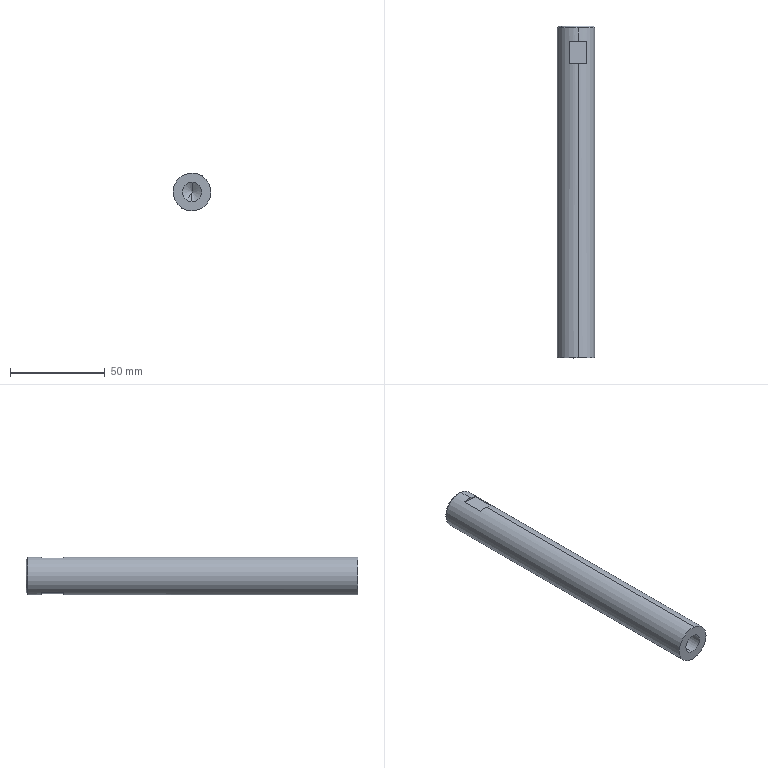Component | SolidWorks | SHYTJ-01-03-06GuideAxis-2 | 1 solid | 16 faces | box 20 x 175 x 20 mm | volume 52333 mm3 | plane 8 | cylinder 4 | cone 4 | commonest cylinder face diameters 10.2 x2 20 x2
build123d program:
from build123d import *

# Parameters (mm, degrees)
SKETCH1_W               = 175
SKETCH1_H               = 10
CHAMFER1_SIZE           = 1
CUT_EXTRUDE2_DEPTH      = 10
CUT_EXTRUDE2_DEPTH_BACK = 10
SKETCH3_W               = 12
SKETCH3_H               = 4.511
SKETCH3_H_2             = 3.871
M12_TAPPED_HOLE2_D      = 10.2
M12_TAPPED_HOLE2_DEPTH  = 29.25
M12_TAPPED_HOLE2_TIP    = 3.064


with BuildPart() as part:
    # Sketch1 → Revolve1 (revolve)
    with BuildSketch(Plane.XY, mode=Mode.PRIVATE) as revolve1_sk:
        with Locations((87.5, 5)):
            Rectangle(SKETCH1_W, SKETCH1_H)
    revolve(revolve1_sk.sketch.rotate(Axis((0, 0, 0), (1, 0, 0)), 90), axis=Axis((0, 0, 0), (1, 0, 0)))

    # Chamfer1
    chamfer1_edges = [part.edges().sort_by_distance(p)[0] for p in [
        (175, 0, -10),
    ]]
    chamfer(chamfer1_edges, length=CHAMFER1_SIZE)

    # Sketch3 → Cut-Extrude2 (cut, two sides: drawn at the far end of the back side and taken through both)
    with BuildSketch(Plane(origin=(0, 0, 0), x_dir=(1, 0, 0), z_dir=(0, 1, 0)).offset(-CUT_EXTRUDE2_DEPTH_BACK)):
        with Locations((161, -11.255)):
            Rectangle(SKETCH3_W, SKETCH3_H)
        with Locations((161, 10.936)):
            Rectangle(SKETCH3_W, SKETCH3_H_2)
    extrude(amount=CUT_EXTRUDE2_DEPTH + CUT_EXTRUDE2_DEPTH_BACK, mode=Mode.SUBTRACT)

    # M12 Tapped Hole2
    with Locations(Plane.ZY):
        with Locations((0, 0)):
            Hole(M12_TAPPED_HOLE2_D / 2, depth=M12_TAPPED_HOLE2_DEPTH)
            with Locations((0, 0, -(M12_TAPPED_HOLE2_DEPTH + M12_TAPPED_HOLE2_TIP / 2))):  # 118° drill point
                Cone(0, M12_TAPPED_HOLE2_D / 2, M12_TAPPED_HOLE2_TIP, mode=Mode.SUBTRACT)


solid = part.part

# Placed as in the assembly
solid = solid.moved(Location((101.884, -48.361, 270), (0, 6.585, 90)))
STEP:
#1=CARTESIAN_POINT('',(3.988,-0.7524,10.43));
#2=VERTEX_POINT('',#1);
#3=CARTESIAN_POINT('',(4.034,-0.7524,10.829));
#4=VERTEX_POINT('',#3);
#5=CARTESIAN_POINT('',(4.011,-0.7524,10.63));
#6=DIRECTION('',(0.,-1.,-0.));
#7=DIRECTION('',(0.1147,0.,0.9934));
#8=AXIS2_PLACEMENT_3D('',#5,#6,#7);
#9=CIRCLE('',#8,0.2008);
#10=EDGE_CURVE('',#2,#4,#9,.T.);
#11=ORIENTED_EDGE('',*,*,#10,.F.);
#12=CARTESIAN_POINT('',(3.988,-1.904,10.43));
#13=VERTEX_POINT('',#12);
#14=CARTESIAN_POINT('',(3.988,-1.904,10.43));
#15=DIRECTION('',(0.,-1.,-0.));
#16=VECTOR('',#15,39.37);
#17=LINE('',#14,#16);
#18=EDGE_CURVE('',#2,#13,#17,.T.);
#19=ORIENTED_EDGE('',*,*,#18,.T.);
#20=CARTESIAN_POINT('',(4.034,-1.904,10.829));
#21=VERTEX_POINT('',#20);
#22=CARTESIAN_POINT('',(4.011,-1.904,10.63));
#23=DIRECTION('',(0.,-1.,-0.));
#24=DIRECTION('',(0.1147,0.,0.9934));
#25=AXIS2_PLACEMENT_3D('',#22,#23,#24);
#26=CIRCLE('',#25,0.2008);
#27=EDGE_CURVE('',#13,#21,#26,.T.);
#28=ORIENTED_EDGE('',*,*,#27,.T.);
#29=CARTESIAN_POINT('',(4.034,-1.904,10.829));
#30=DIRECTION('',(0.,-1.,-0.));
#31=VECTOR('',#30,39.37);
#32=LINE('',#29,#31);
#33=EDGE_CURVE('',#4,#21,#32,.T.);
#34=ORIENTED_EDGE('',*,*,#33,.F.);
#35=EDGE_LOOP('',(#11,#19,#28,#34));
#36=FACE_OUTER_BOUND('',#35,.T.);
#37=CARTESIAN_POINT('',(4.011,-1.904,10.63));
#38=DIRECTION('',(0.,-1.,-0.));
#39=DIRECTION('',(0.1147,0.,0.9934));
#40=AXIS2_PLACEMENT_3D('',#37,#38,#39);
#41=CYLINDRICAL_SURFACE('',#40,0.2008);
#42=ADVANCED_FACE('',(#36),#41,.F.);
#43=CARTESIAN_POINT('',(4.011,-0.6317,10.63));
#44=VERTEX_POINT('',#43);
#45=CARTESIAN_POINT('',(4.034,-0.7524,10.829));
#46=DIRECTION('',(0.09829,-0.515,0.8515));
#47=VECTOR('',#46,39.37);
#48=LINE('',#45,#47);
#49=EDGE_CURVE('',#44,#4,#48,.T.);
#50=ORIENTED_EDGE('',*,*,#49,.F.);
#51=CARTESIAN_POINT('',(3.988,-0.7524,10.43));
#52=DIRECTION('',(-0.09829,-0.515,-0.8515));
#53=VECTOR('',#52,39.37);
#54=LINE('',#51,#53);
#55=EDGE_CURVE('',#44,#2,#54,.T.);
#56=ORIENTED_EDGE('',*,*,#55,.T.);
#57=ORIENTED_EDGE('',*,*,#10,.T.);
#58=EDGE_LOOP('',(#50,#56,#57));
#59=FACE_OUTER_BOUND('',#58,.T.);
#60=CARTESIAN_POINT('',(4.011,-0.7524,10.63));
#61=DIRECTION('',(0.,-1.,-0.));
#62=DIRECTION('',(0.1147,0.,0.9934));
#63=AXIS2_PLACEMENT_3D('',#60,#61,#62);
#64=CONICAL_SURFACE('',#63,0.2008,1.03);
#65=ADVANCED_FACE('',(#59),#64,.F.);
#66=CARTESIAN_POINT('',(3.971,4.986,10.278));
#67=VERTEX_POINT('',#66);
#68=CARTESIAN_POINT('',(4.052,4.986,10.982));
#69=VERTEX_POINT('',#68);
#70=CARTESIAN_POINT('',(4.011,4.986,10.63));
#71=DIRECTION('',(-0.,1.,0.));
#72=DIRECTION('',(0.1147,0.,0.9934));
#73=AXIS2_PLACEMENT_3D('',#70,#71,#72);
#74=CIRCLE('',#73,0.3543);
#75=EDGE_CURVE('',#67,#69,#74,.T.);
#76=ORIENTED_EDGE('',*,*,#75,.F.);
#77=CARTESIAN_POINT('',(3.966,4.946,10.239));
#78=VERTEX_POINT('',#77);
#79=CARTESIAN_POINT('',(3.966,4.946,10.239));
#80=DIRECTION('',(-0.08109,-0.7071,-0.7024));
#81=VECTOR('',#80,39.37);
#82=LINE('',#79,#81);
#83=EDGE_CURVE('',#67,#78,#82,.T.);
#84=ORIENTED_EDGE('',*,*,#83,.T.);
#85=CARTESIAN_POINT('',(4.056,4.946,11.021));
#86=VERTEX_POINT('',#85);
#87=CARTESIAN_POINT('',(4.011,4.946,10.63));
#88=DIRECTION('',(0.,-1.,-0.));
#89=DIRECTION('',(0.1147,0.,0.9934));
#90=AXIS2_PLACEMENT_3D('',#87,#88,#89);
#91=CIRCLE('',#90,0.3937);
#92=EDGE_CURVE('',#86,#78,#91,.T.);
#93=ORIENTED_EDGE('',*,*,#92,.F.);
#94=CARTESIAN_POINT('',(4.056,4.946,11.021));
#95=DIRECTION('',(0.08109,-0.7071,0.7024));
#96=VECTOR('',#95,39.37);
#97=LINE('',#94,#96);
#98=EDGE_CURVE('',#69,#86,#97,.T.);
#99=ORIENTED_EDGE('',*,*,#98,.F.);
#100=EDGE_LOOP('',(#76,#84,#93,#99));
#101=FACE_OUTER_BOUND('',#100,.T.);
#102=CARTESIAN_POINT('',(4.011,4.946,10.63));
#103=DIRECTION('',(0.,-1.,-0.));
#104=DIRECTION('',(0.1147,0.,0.9934));
#105=AXIS2_PLACEMENT_3D('',#102,#103,#104);
#106=CONICAL_SURFACE('',#105,0.3937,0.7854);
#107=ADVANCED_FACE('',(#101),#106,.T.);
#108=ORIENTED_EDGE('',*,*,#92,.T.);
#109=CARTESIAN_POINT('',(3.966,4.671,10.239));
#110=VERTEX_POINT('',#109);
#111=CARTESIAN_POINT('',(3.966,-1.904,10.239));
#112=DIRECTION('',(0.,-1.,-0.));
#113=VECTOR('',#112,39.37);
#114=LINE('',#111,#113);
#115=EDGE_CURVE('',#78,#110,#114,.T.);
#116=ORIENTED_EDGE('',*,*,#115,.T.);
#117=CARTESIAN_POINT('',(3.8,4.671,10.298));
#118=VERTEX_POINT('',#117);
#119=CARTESIAN_POINT('',(4.011,4.671,10.63));
#120=DIRECTION('',(0.,-1.,-0.));
#121=DIRECTION('',(0.1147,0.,0.9934));
#122=AXIS2_PLACEMENT_3D('',#119,#120,#121);
#123=CIRCLE('',#122,0.3937);
#124=EDGE_CURVE('',#118,#110,#123,.T.);
#125=ORIENTED_EDGE('',*,*,#124,.F.);
#126=CARTESIAN_POINT('',(3.8,4.198,10.298));
#127=VERTEX_POINT('',#126);
#128=CARTESIAN_POINT('',(3.8,-1.904,10.298));
#129=DIRECTION('',(-0.,1.,0.));
#130=VECTOR('',#129,39.37);
#131=LINE('',#128,#130);
#132=EDGE_CURVE('',#127,#118,#131,.T.);
#133=ORIENTED_EDGE('',*,*,#132,.F.);
#134=CARTESIAN_POINT('',(3.966,4.198,10.239));
#135=VERTEX_POINT('',#134);
#136=CARTESIAN_POINT('',(4.011,4.198,10.63));
#137=DIRECTION('',(-0.,1.,0.));
#138=DIRECTION('',(-0.1147,0.,-0.9934));
#139=AXIS2_PLACEMENT_3D('',#136,#137,#138);
#140=CIRCLE('',#139,0.3937);
#141=EDGE_CURVE('',#135,#127,#140,.T.);
#142=ORIENTED_EDGE('',*,*,#141,.F.);
#143=CARTESIAN_POINT('',(3.966,-1.904,10.239));
#144=VERTEX_POINT('',#143);
#145=CARTESIAN_POINT('',(3.966,-1.904,10.239));
#146=DIRECTION('',(0.,-1.,-0.));
#147=VECTOR('',#146,39.37);
#148=LINE('',#145,#147);
#149=EDGE_CURVE('',#135,#144,#148,.T.);
#150=ORIENTED_EDGE('',*,*,#149,.T.);
#151=CARTESIAN_POINT('',(4.056,-1.904,11.021));
#152=VERTEX_POINT('',#151);
#153=CARTESIAN_POINT('',(4.011,-1.904,10.63));
#154=DIRECTION('',(0.,-1.,-0.));
#155=DIRECTION('',(0.1147,0.,0.9934));
#156=AXIS2_PLACEMENT_3D('',#153,#154,#155);
#157=CIRCLE('',#156,0.3937);
#158=EDGE_CURVE('',#152,#144,#157,.T.);
#159=ORIENTED_EDGE('',*,*,#158,.F.);
#160=CARTESIAN_POINT('',(4.056,4.198,11.021));
#161=VERTEX_POINT('',#160);
#162=CARTESIAN_POINT('',(4.056,-1.904,11.021));
#163=DIRECTION('',(0.,-1.,-0.));
#164=VECTOR('',#163,39.37);
#165=LINE('',#162,#164);
#166=EDGE_CURVE('',#161,#152,#165,.T.);
#167=ORIENTED_EDGE('',*,*,#166,.F.);
#168=CARTESIAN_POINT('',(3.881,4.198,11.002));
#169=VERTEX_POINT('',#168);
#170=CARTESIAN_POINT('',(4.011,4.198,10.63));
#171=DIRECTION('',(-0.,1.,0.));
#172=DIRECTION('',(-0.1147,0.,-0.9934));
#173=AXIS2_PLACEMENT_3D('',#170,#171,#172);
#174=CIRCLE('',#173,0.3937);
#175=EDGE_CURVE('',#169,#161,#174,.T.);
#176=ORIENTED_EDGE('',*,*,#175,.F.);
#177=CARTESIAN_POINT('',(3.881,4.671,11.002));
#178=VERTEX_POINT('',#177);
#179=CARTESIAN_POINT('',(3.881,-1.904,11.002));
#180=DIRECTION('',(0.,-1.,-0.));
#181=VECTOR('',#180,39.37);
#182=LINE('',#179,#181);
#183=EDGE_CURVE('',#178,#169,#182,.T.);
#184=ORIENTED_EDGE('',*,*,#183,.F.);
#185=CARTESIAN_POINT('',(4.056,4.671,11.021));
#186=VERTEX_POINT('',#185);
#187=CARTESIAN_POINT('',(4.011,4.671,10.63));
#188=DIRECTION('',(0.,-1.,-0.));
#189=DIRECTION('',(0.1147,0.,0.9934));
#190=AXIS2_PLACEMENT_3D('',#187,#188,#189);
#191=CIRCLE('',#190,0.3937);
#192=EDGE_CURVE('',#186,#178,#191,.T.);
#193=ORIENTED_EDGE('',*,*,#192,.F.);
#194=CARTESIAN_POINT('',(4.056,-1.904,11.021));
#195=DIRECTION('',(0.,-1.,-0.));
#196=VECTOR('',#195,39.37);
#197=LINE('',#194,#196);
#198=EDGE_CURVE('',#86,#186,#197,.T.);
#199=ORIENTED_EDGE('',*,*,#198,.F.);
#200=EDGE_LOOP('',(#108,#116,#125,#133,#142,#150,#159,#167,#176,#184,#193,#199));
#201=FACE_OUTER_BOUND('',#200,.T.);
#202=CARTESIAN_POINT('',(4.011,-1.904,10.63));
#203=DIRECTION('',(0.,-1.,-0.));
#204=DIRECTION('',(0.1147,0.,0.9934));
#205=AXIS2_PLACEMENT_3D('',#202,#203,#204);
#206=CYLINDRICAL_SURFACE('',#205,0.3937);
#207=ADVANCED_FACE('',(#201),#206,.T.);
#208=ORIENTED_EDGE('',*,*,#115,.F.);
#209=CARTESIAN_POINT('',(4.011,4.946,10.63));
#210=DIRECTION('',(0.,-1.,-0.));
#211=DIRECTION('',(0.1147,0.,0.9934));
#212=AXIS2_PLACEMENT_3D('',#209,#210,#211);
#213=CIRCLE('',#212,0.3937);
#214=EDGE_CURVE('',#78,#86,#213,.T.);
#215=ORIENTED_EDGE('',*,*,#214,.T.);
#216=ORIENTED_EDGE('',*,*,#198,.T.);
#217=CARTESIAN_POINT('',(4.222,4.671,10.962));
#218=VERTEX_POINT('',#217);
#219=CARTESIAN_POINT('',(4.011,4.671,10.63));
#220=DIRECTION('',(0.,-1.,-0.));
#221=DIRECTION('',(0.1147,0.,0.9934));
#222=AXIS2_PLACEMENT_3D('',#219,#220,#221);
#223=CIRCLE('',#222,0.3937);
#224=EDGE_CURVE('',#218,#186,#223,.T.);
#225=ORIENTED_EDGE('',*,*,#224,.F.);
#226=CARTESIAN_POINT('',(4.222,4.198,10.962));
#227=VERTEX_POINT('',#226);
#228=CARTESIAN_POINT('',(4.222,-1.904,10.962));
#229=DIRECTION('',(-0.,1.,0.));
#230=VECTOR('',#229,39.37);
#231=LINE('',#228,#230);
#232=EDGE_CURVE('',#227,#218,#231,.T.);
#233=ORIENTED_EDGE('',*,*,#232,.F.);
#234=CARTESIAN_POINT('',(4.011,4.198,10.63));
#235=DIRECTION('',(-0.,1.,0.));
#236=DIRECTION('',(-0.1147,0.,-0.9934));
#237=AXIS2_PLACEMENT_3D('',#234,#235,#236);
#238=CIRCLE('',#237,0.3937);
#239=EDGE_CURVE('',#161,#227,#238,.T.);
#240=ORIENTED_EDGE('',*,*,#239,.F.);
#241=ORIENTED_EDGE('',*,*,#166,.T.);
#242=CARTESIAN_POINT('',(4.011,-1.904,10.63));
#243=DIRECTION('',(0.,-1.,-0.));
#244=DIRECTION('',(0.1147,0.,0.9934));
#245=AXIS2_PLACEMENT_3D('',#242,#243,#244);
#246=CIRCLE('',#245,0.3937);
#247=EDGE_CURVE('',#144,#152,#246,.T.);
#248=ORIENTED_EDGE('',*,*,#247,.F.);
#249=ORIENTED_EDGE('',*,*,#149,.F.);
#250=CARTESIAN_POINT('',(4.141,4.198,10.258));
#251=VERTEX_POINT('',#250);
#252=CARTESIAN_POINT('',(4.011,4.198,10.63));
#253=DIRECTION('',(-0.,1.,0.));
#254=DIRECTION('',(-0.1147,0.,-0.9934));
#255=AXIS2_PLACEMENT_3D('',#252,#253,#254);
#256=CIRCLE('',#255,0.3937);
#257=EDGE_CURVE('',#251,#135,#256,.T.);
#258=ORIENTED_EDGE('',*,*,#257,.F.);
#259=CARTESIAN_POINT('',(4.141,4.671,10.258));
#260=VERTEX_POINT('',#259);
#261=CARTESIAN_POINT('',(4.141,-1.904,10.258));
#262=DIRECTION('',(0.,-1.,-0.));
#263=VECTOR('',#262,39.37);
#264=LINE('',#261,#263);
#265=EDGE_CURVE('',#260,#251,#264,.T.);
#266=ORIENTED_EDGE('',*,*,#265,.F.);
#267=CARTESIAN_POINT('',(4.011,4.671,10.63));
#268=DIRECTION('',(0.,-1.,-0.));
#269=DIRECTION('',(0.1147,0.,0.9934));
#270=AXIS2_PLACEMENT_3D('',#267,#268,#269);
#271=CIRCLE('',#270,0.3937);
#272=EDGE_CURVE('',#110,#260,#271,.T.);
#273=ORIENTED_EDGE('',*,*,#272,.F.);
#274=EDGE_LOOP('',(#208,#215,#216,#225,#233,#240,#241,#248,#249,#258,#266,#273));
#275=FACE_OUTER_BOUND('',#274,.T.);
#276=CARTESIAN_POINT('',(4.011,-1.904,10.63));
#277=DIRECTION('',(0.,-1.,-0.));
#278=DIRECTION('',(0.1147,0.,0.9934));
#279=AXIS2_PLACEMENT_3D('',#276,#277,#278);
#280=CYLINDRICAL_SURFACE('',#279,0.3937);
#281=ADVANCED_FACE('',(#275),#280,.T.);
#282=CARTESIAN_POINT('',(4.011,-1.904,10.63));
#283=DIRECTION('',(0.,-1.,-0.));
#284=DIRECTION('',(0.1147,0.,0.9934));
#285=AXIS2_PLACEMENT_3D('',#282,#283,#284);
#286=CIRCLE('',#285,0.2008);
#287=EDGE_CURVE('',#21,#13,#286,.T.);
#288=ORIENTED_EDGE('',*,*,#287,.F.);
#289=ORIENTED_EDGE('',*,*,#27,.F.);
#290=EDGE_LOOP('',(#288,#289));
#291=FACE_BOUND('',#290,.T.);
#292=ORIENTED_EDGE('',*,*,#158,.T.);
#293=ORIENTED_EDGE('',*,*,#247,.T.);
#294=EDGE_LOOP('',(#292,#293));
#295=FACE_OUTER_BOUND('',#294,.T.);
#296=CARTESIAN_POINT('',(4.011,-1.904,10.63));
#297=DIRECTION('',(-0.,1.,0.));
#298=DIRECTION('',(-0.1147,0.,-0.9934));
#299=AXIS2_PLACEMENT_3D('',#296,#297,#298);
#300=PLANE('',#299);
#301=ADVANCED_FACE('',(#291,#295),#300,.F.);
#302=CARTESIAN_POINT('',(4.011,4.986,10.63));
#303=DIRECTION('',(-0.,1.,0.));
#304=DIRECTION('',(0.1147,0.,0.9934));
#305=AXIS2_PLACEMENT_3D('',#302,#303,#304);
#306=CIRCLE('',#305,0.3543);
#307=EDGE_CURVE('',#69,#67,#306,.T.);
#308=ORIENTED_EDGE('',*,*,#307,.T.);
#309=ORIENTED_EDGE('',*,*,#75,.T.);
#310=EDGE_LOOP('',(#308,#309));
#311=FACE_OUTER_BOUND('',#310,.T.);
#312=CARTESIAN_POINT('',(4.011,4.986,10.63));
#313=DIRECTION('',(0.,-1.,-0.));
#314=DIRECTION('',(0.1147,-0.,0.9934));
#315=AXIS2_PLACEMENT_3D('',#312,#313,#314);
#316=PLANE('',#315);
#317=ADVANCED_FACE('',(#311),#316,.F.);
#318=ORIENTED_EDGE('',*,*,#83,.F.);
#319=ORIENTED_EDGE('',*,*,#307,.F.);
#320=ORIENTED_EDGE('',*,*,#98,.T.);
#321=ORIENTED_EDGE('',*,*,#214,.F.);
#322=EDGE_LOOP('',(#318,#319,#320,#321));
#323=FACE_OUTER_BOUND('',#322,.T.);
#324=CARTESIAN_POINT('',(4.011,4.946,10.63));
#325=DIRECTION('',(0.,-1.,-0.));
#326=DIRECTION('',(0.1147,0.,0.9934));
#327=AXIS2_PLACEMENT_3D('',#324,#325,#326);
#328=CONICAL_SURFACE('',#327,0.3937,0.7854);
#329=ADVANCED_FACE('',(#323),#328,.T.);
#330=ORIENTED_EDGE('',*,*,#224,.T.);
#331=ORIENTED_EDGE('',*,*,#192,.T.);
#332=CARTESIAN_POINT('',(3.661,4.671,11.027));
#333=DIRECTION('',(0.9934,0.,-0.1147));
#334=VECTOR('',#333,39.37);
#335=LINE('',#332,#334);
#336=EDGE_CURVE('',#178,#218,#335,.T.);
#337=ORIENTED_EDGE('',*,*,#336,.T.);
#338=EDGE_LOOP('',(#330,#331,#337));
#339=FACE_OUTER_BOUND('',#338,.T.);
#340=CARTESIAN_POINT('',(3.661,4.671,11.027));
#341=DIRECTION('',(0.,-1.,-0.));
#342=DIRECTION('',(0.1147,-0.,0.9934));
#343=AXIS2_PLACEMENT_3D('',#340,#341,#342);
#344=PLANE('',#343);
#345=ADVANCED_FACE('',(#339),#344,.T.);
#346=ORIENTED_EDGE('',*,*,#183,.T.);
#347=CARTESIAN_POINT('',(3.661,4.198,11.027));
#348=DIRECTION('',(0.9934,0.,-0.1147));
#349=VECTOR('',#348,39.37);
#350=LINE('',#347,#349);
#351=EDGE_CURVE('',#169,#227,#350,.T.);
#352=ORIENTED_EDGE('',*,*,#351,.T.);
#353=ORIENTED_EDGE('',*,*,#232,.T.);
#354=ORIENTED_EDGE('',*,*,#336,.F.);
#355=EDGE_LOOP('',(#346,#352,#353,#354));
#356=FACE_OUTER_BOUND('',#355,.T.);
#357=CARTESIAN_POINT('',(3.661,4.671,11.027));
#358=DIRECTION('',(0.1147,-0.,0.9934));
#359=DIRECTION('',(-0.,1.,0.));
#360=AXIS2_PLACEMENT_3D('',#357,#358,#359);
#361=PLANE('',#360);
#362=ADVANCED_FACE('',(#356),#361,.T.);
#363=ORIENTED_EDGE('',*,*,#175,.T.);
#364=ORIENTED_EDGE('',*,*,#239,.T.);
#365=ORIENTED_EDGE('',*,*,#351,.F.);
#366=EDGE_LOOP('',(#363,#364,#365));
#367=FACE_OUTER_BOUND('',#366,.T.);
#368=CARTESIAN_POINT('',(3.661,4.198,11.027));
#369=DIRECTION('',(-0.,1.,0.));
#370=DIRECTION('',(-0.1147,0.,-0.9934));
#371=AXIS2_PLACEMENT_3D('',#368,#369,#370);
#372=PLANE('',#371);
#373=ADVANCED_FACE('',(#367),#372,.T.);
#374=ORIENTED_EDGE('',*,*,#257,.T.);
#375=ORIENTED_EDGE('',*,*,#141,.T.);
#376=CARTESIAN_POINT('',(3.579,4.198,10.323));
#377=DIRECTION('',(0.9934,0.,-0.1147));
#378=VECTOR('',#377,39.37);
#379=LINE('',#376,#378);
#380=EDGE_CURVE('',#127,#251,#379,.T.);
#381=ORIENTED_EDGE('',*,*,#380,.T.);
#382=EDGE_LOOP('',(#374,#375,#381));
#383=FACE_OUTER_BOUND('',#382,.T.);
#384=CARTESIAN_POINT('',(3.562,4.198,10.172));
#385=DIRECTION('',(-0.,1.,0.));
#386=DIRECTION('',(-0.1147,0.,-0.9934));
#387=AXIS2_PLACEMENT_3D('',#384,#385,#386);
#388=PLANE('',#387);
#389=ADVANCED_FACE('',(#383),#388,.T.);
#390=ORIENTED_EDGE('',*,*,#265,.T.);
#391=ORIENTED_EDGE('',*,*,#380,.F.);
#392=ORIENTED_EDGE('',*,*,#132,.T.);
#393=CARTESIAN_POINT('',(3.579,4.671,10.323));
#394=DIRECTION('',(0.9934,0.,-0.1147));
#395=VECTOR('',#394,39.37);
#396=LINE('',#393,#395);
#397=EDGE_CURVE('',#118,#260,#396,.T.);
#398=ORIENTED_EDGE('',*,*,#397,.T.);
#399=EDGE_LOOP('',(#390,#391,#392,#398));
#400=FACE_OUTER_BOUND('',#399,.T.);
#401=CARTESIAN_POINT('',(3.579,4.198,10.323));
#402=DIRECTION('',(-0.1147,-0.,-0.9934));
#403=DIRECTION('',(0.,-1.,0.));
#404=AXIS2_PLACEMENT_3D('',#401,#402,#403);
#405=PLANE('',#404);
#406=ADVANCED_FACE('',(#400),#405,.T.);
#407=ORIENTED_EDGE('',*,*,#124,.T.);
#408=ORIENTED_EDGE('',*,*,#272,.T.);
#409=ORIENTED_EDGE('',*,*,#397,.F.);
#410=EDGE_LOOP('',(#407,#408,#409));
#411=FACE_OUTER_BOUND('',#410,.T.);
#412=CARTESIAN_POINT('',(3.562,4.671,10.172));
#413=DIRECTION('',(0.,-1.,-0.));
#414=DIRECTION('',(0.1147,-0.,0.9934));
#415=AXIS2_PLACEMENT_3D('',#412,#413,#414);
#416=PLANE('',#415);
#417=ADVANCED_FACE('',(#411),#416,.T.);
#418=ORIENTED_EDGE('',*,*,#55,.F.);
#419=ORIENTED_EDGE('',*,*,#49,.T.);
#420=CARTESIAN_POINT('',(4.011,-0.7524,10.63));
#421=DIRECTION('',(0.,-1.,-0.));
#422=DIRECTION('',(0.1147,0.,0.9934));
#423=AXIS2_PLACEMENT_3D('',#420,#421,#422);
#424=CIRCLE('',#423,0.2008);
#425=EDGE_CURVE('',#4,#2,#424,.T.);
#426=ORIENTED_EDGE('',*,*,#425,.T.);
#427=EDGE_LOOP('',(#418,#419,#426));
#428=FACE_OUTER_BOUND('',#427,.T.);
#429=CARTESIAN_POINT('',(4.011,-0.7524,10.63));
#430=DIRECTION('',(0.,-1.,-0.));
#431=DIRECTION('',(0.1147,0.,0.9934));
#432=AXIS2_PLACEMENT_3D('',#429,#430,#431);
#433=CONICAL_SURFACE('',#432,0.2008,1.03);
#434=ADVANCED_FACE('',(#428),#433,.F.);
#435=ORIENTED_EDGE('',*,*,#18,.F.);
#436=ORIENTED_EDGE('',*,*,#425,.F.);
#437=ORIENTED_EDGE('',*,*,#33,.T.);
#438=ORIENTED_EDGE('',*,*,#287,.T.);
#439=EDGE_LOOP('',(#435,#436,#437,#438));
#440=FACE_OUTER_BOUND('',#439,.T.);
#441=CARTESIAN_POINT('',(4.011,-1.904,10.63));
#442=DIRECTION('',(0.,-1.,-0.));
#443=DIRECTION('',(0.1147,0.,0.9934));
#444=AXIS2_PLACEMENT_3D('',#441,#442,#443);
#445=CYLINDRICAL_SURFACE('',#444,0.2008);
#446=ADVANCED_FACE('',(#440),#445,.F.);
#447=CLOSED_SHELL('',(#42,#65,#107,#207,#281,#301,#317,#329,#345,#362,#373,#389,#406,#417,#434,#446));
#448=MANIFOLD_SOLID_BREP('',#447);
#449=CARTESIAN_POINT('',(0.,0.,0.));
#450=DIRECTION('',(0.,0.,1.));
#451=DIRECTION('',(1.,0.,0.));
#452=AXIS2_PLACEMENT_3D('',#449,#450,#451);
#453=(LENGTH_UNIT()NAMED_UNIT(*)SI_UNIT($,.METRE.));
#454=LENGTH_MEASURE_WITH_UNIT(LENGTH_MEASURE(0.0254),#453);
#455=DIMENSIONAL_EXPONENTS(1.,0.,0.,0.,0.,0.,0.);
#456=(CONVERSION_BASED_UNIT('',#454)LENGTH_UNIT()NAMED_UNIT(#455));
#457=UNCERTAINTY_MEASURE_WITH_UNIT(LENGTH_MEASURE(0.00001),#456,'','');
#458=(NAMED_UNIT(*)PLANE_ANGLE_UNIT()SI_UNIT($,.RADIAN.));
#459=(NAMED_UNIT(*)SI_UNIT($,.STERADIAN.)SOLID_ANGLE_UNIT());
#460=(GEOMETRIC_REPRESENTATION_CONTEXT(3)GLOBAL_UNCERTAINTY_ASSIGNED_CONTEXT((#457))GLOBAL_UNIT_ASSIGNED_CONTEXT((#456,#458,#459))REPRESENTATION_CONTEXT('',''));
#461=ADVANCED_BREP_SHAPE_REPRESENTATION('',(#448,#452),#460);
#462=COLOUR_RGB('',0.7922,0.8196,0.9333);
#463=FILL_AREA_STYLE_COLOUR('',#462);
#464=FILL_AREA_STYLE('',(#463));
#465=SURFACE_STYLE_FILL_AREA(#464);
#466=SURFACE_SIDE_STYLE('',(#465));
#467=SURFACE_STYLE_USAGE(.BOTH.,#466);
#468=PRESENTATION_STYLE_ASSIGNMENT((#467));
#469=STYLED_ITEM('',(#468),#448);
#470=(LENGTH_UNIT()NAMED_UNIT(*)SI_UNIT($,.METRE.));
#471=LENGTH_MEASURE_WITH_UNIT(LENGTH_MEASURE(0.0254),#470);
#472=DIMENSIONAL_EXPONENTS(1.,0.,0.,0.,0.,0.,0.);
#473=(CONVERSION_BASED_UNIT('',#471)LENGTH_UNIT()NAMED_UNIT(#472));
#474=UNCERTAINTY_MEASURE_WITH_UNIT(LENGTH_MEASURE(0.00001),#473,'','');
#475=(NAMED_UNIT(*)PLANE_ANGLE_UNIT()SI_UNIT($,.RADIAN.));
#476=(NAMED_UNIT(*)SI_UNIT($,.STERADIAN.)SOLID_ANGLE_UNIT());
#477=(GEOMETRIC_REPRESENTATION_CONTEXT(3)GLOBAL_UNCERTAINTY_ASSIGNED_CONTEXT((#474))GLOBAL_UNIT_ASSIGNED_CONTEXT((#473,#475,#476))REPRESENTATION_CONTEXT('',''));
#478=MECHANICAL_DESIGN_GEOMETRIC_PRESENTATION_REPRESENTATION('',(#469),#477);
#479=PRESENTATION_LAYER_ASSIGNMENT('','',(#469));